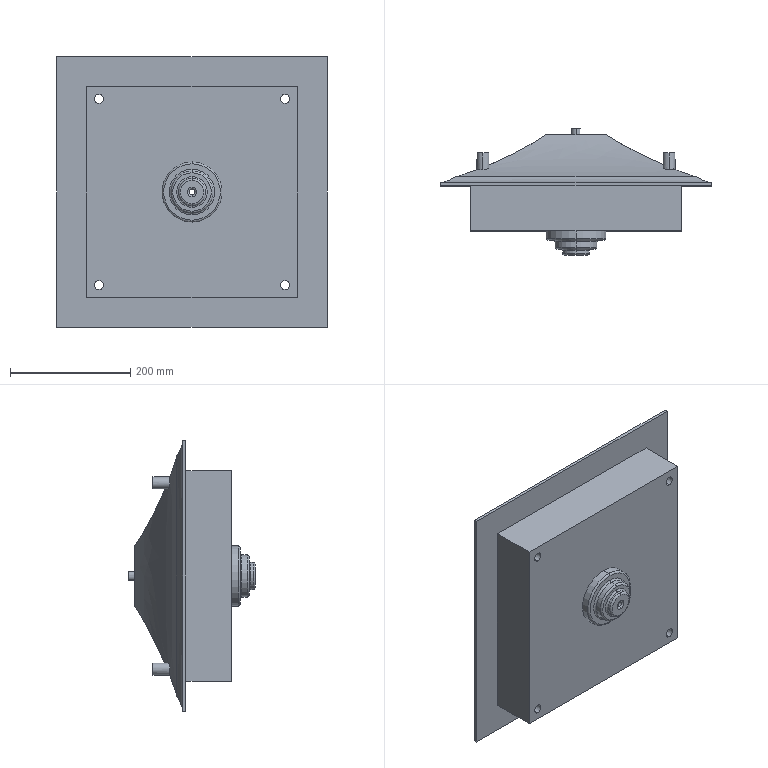Component | SolidWorks | InsectTrapLamp-1_InsectTrapLampTop-1 | 1 solid | 65 faces | volume 16374871 mm3 | cylinder 26 | plane 19 | torus 12 | spline 8 | commonest cylinder face diameters 15 x10 20 x8 45 x2 70 x2 100 x2 10 x2